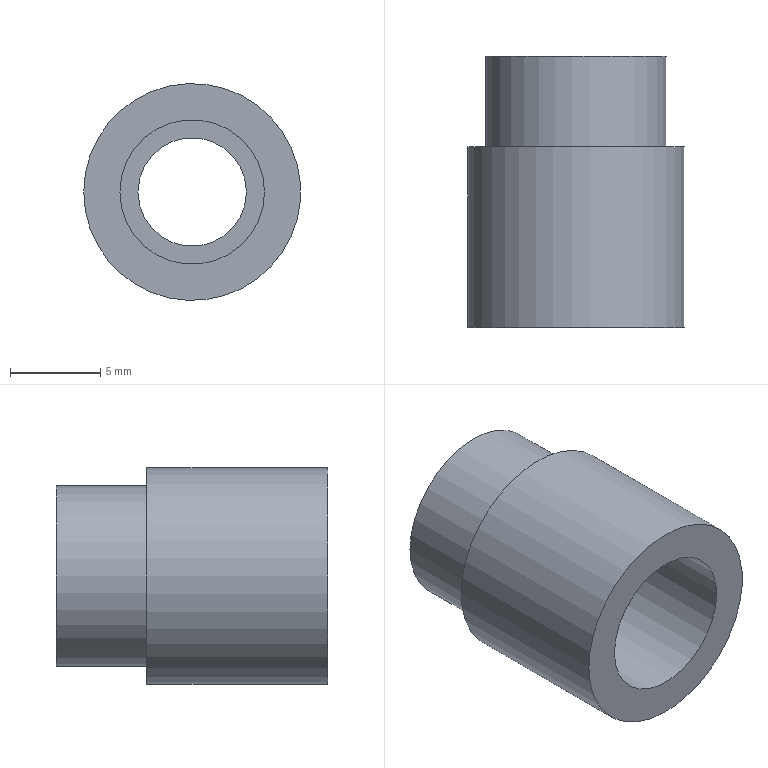Component | NX | 05D__27_2 | 1 solid | 8 faces | box 12 x 15 x 12 mm | volume 924 mm3 | cylinder 4 | plane 4 | commonest cylinder face diameters 6 x1 10 x1 12 x1 8 x1
STEP:
#1=CARTESIAN_POINT('',(0.,0.,0.));
#2=DIRECTION('',(0.,0.,1.));
#3=DIRECTION('',(1.,0.,0.));
#4=AXIS2_PLACEMENT_3D('',#1,#2,#3);
#5=CARTESIAN_POINT('',(63.522,90.09,209.432));
#6=VERTEX_POINT('',#5);
#7=CARTESIAN_POINT('',(66.522,90.09,209.432));
#8=DIRECTION('',(0.,1.,0.));
#9=DIRECTION('',(-1.,0.,0.));
#10=AXIS2_PLACEMENT_3D('',#7,#8,#9);
#11=CIRCLE('',#10,3.);
#12=CARTESIAN_POINT('',(66.522,90.09,209.432));
#13=DIRECTION('',(0.,1.,0.));
#14=DIRECTION('',(-1.,0.,0.));
#15=AXIS2_PLACEMENT_3D('',#12,#13,#14);
#16=CYLINDRICAL_SURFACE('',#15,3.);
#17=CARTESIAN_POINT('',(0.,0.));
#18=DIRECTION('',(1.,0.));
#19=VECTOR('',#18,1.);
#20=LINE('',#17,#19);
#21=(GEOMETRIC_REPRESENTATION_CONTEXT(2)PARAMETRIC_REPRESENTATION_CONTEXT()REPRESENTATION_CONTEXT('',''));
#22=DEFINITIONAL_REPRESENTATION('',(#20),#21);
#23=PCURVE('',#16,#22);
#24=CARTESIAN_POINT('',(66.522,90.09,212.432));
#25=DIRECTION('',(0.,1.,0.));
#26=DIRECTION('',(-1.,0.,0.));
#27=AXIS2_PLACEMENT_3D('',#24,#25,#26);
#28=PLANE('',#27);
#29=CARTESIAN_POINT('',(0.,-3.));
#30=DIRECTION('',(1.,0.));
#31=AXIS2_PLACEMENT_2D('',#29,#30);
#32=CIRCLE('',#31,3.);
#33=(GEOMETRIC_REPRESENTATION_CONTEXT(2)PARAMETRIC_REPRESENTATION_CONTEXT()REPRESENTATION_CONTEXT('',''));
#34=DEFINITIONAL_REPRESENTATION('',(#32),#33);
#35=PCURVE('',#28,#34);
#36=SURFACE_CURVE('',#11,(#23,#35),.PCURVE_S1.);
#37=EDGE_CURVE('',#6,#6,#36,.T.);
#38=ORIENTED_EDGE('',*,*,#37,.F.);
#39=CARTESIAN_POINT('',(63.522,83.09,209.432));
#40=VERTEX_POINT('',#39);
#41=CARTESIAN_POINT('',(63.522,83.09,209.432));
#42=CARTESIAN_POINT('',(63.522,90.09,209.432));
#43=B_SPLINE_CURVE_WITH_KNOTS('',1,(#41,#42),.UNSPECIFIED.,.F.,.F.,(2,2),(-7.,0.),.PIECEWISE_BEZIER_KNOTS.);
#44=CARTESIAN_POINT('',(0.,0.));
#45=DIRECTION('',(0.,1.));
#46=VECTOR('',#45,1.);
#47=LINE('',#44,#46);
#48=(GEOMETRIC_REPRESENTATION_CONTEXT(2)PARAMETRIC_REPRESENTATION_CONTEXT()REPRESENTATION_CONTEXT('',''));
#49=DEFINITIONAL_REPRESENTATION('',(#47),#48);
#50=PCURVE('',#16,#49);
#51=CARTESIAN_POINT('',(6.283,0.));
#52=DIRECTION('',(0.,1.));
#53=VECTOR('',#52,1.);
#54=LINE('',#51,#53);
#55=(GEOMETRIC_REPRESENTATION_CONTEXT(2)PARAMETRIC_REPRESENTATION_CONTEXT()REPRESENTATION_CONTEXT('',''));
#56=DEFINITIONAL_REPRESENTATION('',(#54),#55);
#57=PCURVE('',#16,#56);
#58=SEAM_CURVE('',#43,(#50,#57),.PCURVE_S1.);
#59=EDGE_CURVE('',#40,#6,#58,.T.);
#60=ORIENTED_EDGE('',*,*,#59,.F.);
#61=CARTESIAN_POINT('',(66.522,83.09,209.432));
#62=DIRECTION('',(0.,1.,0.));
#63=DIRECTION('',(-1.,0.,0.));
#64=AXIS2_PLACEMENT_3D('',#61,#62,#63);
#65=CIRCLE('',#64,3.);
#66=CARTESIAN_POINT('',(0.,-7.));
#67=DIRECTION('',(1.,0.));
#68=VECTOR('',#67,1.);
#69=LINE('',#66,#68);
#70=(GEOMETRIC_REPRESENTATION_CONTEXT(2)PARAMETRIC_REPRESENTATION_CONTEXT()REPRESENTATION_CONTEXT('',''));
#71=DEFINITIONAL_REPRESENTATION('',(#69),#70);
#72=PCURVE('',#16,#71);
#73=CARTESIAN_POINT('',(66.522,83.09,213.432));
#74=DIRECTION('',(0.,-1.,-0.));
#75=DIRECTION('',(1.,0.,0.));
#76=AXIS2_PLACEMENT_3D('',#73,#74,#75);
#77=PLANE('',#76);
#78=CARTESIAN_POINT('',(-3.,-4.));
#79=CARTESIAN_POINT('',(-3.,1.196));
#80=CARTESIAN_POINT('',(1.5,-1.402));
#81=CARTESIAN_POINT('',(6.,-4.));
#82=CARTESIAN_POINT('',(1.5,-6.598));
#83=CARTESIAN_POINT('',(-3.,-9.196));
#84=CARTESIAN_POINT('',(-3.,-4.));
#85=(BOUNDED_CURVE()B_SPLINE_CURVE(2,(#78,#79,#80,#81,#82,#83,#84),.UNSPECIFIED.,.T.,.F.)B_SPLINE_CURVE_WITH_KNOTS((1,2,2,2,2,1),(-2.094,0.,2.094,4.189,6.283,8.378),.UNSPECIFIED.)CURVE()GEOMETRIC_REPRESENTATION_ITEM()RATIONAL_B_SPLINE_CURVE((1.,0.5,1.,0.5,1.,0.5,1.))REPRESENTATION_ITEM(''));
#86=(GEOMETRIC_REPRESENTATION_CONTEXT(2)PARAMETRIC_REPRESENTATION_CONTEXT()REPRESENTATION_CONTEXT('',''));
#87=DEFINITIONAL_REPRESENTATION('',(#85),#86);
#88=PCURVE('',#77,#87);
#89=SURFACE_CURVE('',#65,(#72,#88),.PCURVE_S1.);
#90=EDGE_CURVE('',#40,#40,#89,.T.);
#91=ORIENTED_EDGE('',*,*,#90,.T.);
#92=ORIENTED_EDGE('',*,*,#59,.T.);
#93=EDGE_LOOP('',(#38,#60,#91,#92));
#94=FACE_BOUND('',#93,.F.);
#95=ADVANCED_FACE('',(#94),#16,.F.);
#96=CARTESIAN_POINT('',(61.522,90.09,209.432));
#97=VERTEX_POINT('',#96);
#98=CARTESIAN_POINT('',(66.522,90.09,209.432));
#99=DIRECTION('',(0.,1.,0.));
#100=DIRECTION('',(-1.,0.,0.));
#101=AXIS2_PLACEMENT_3D('',#98,#99,#100);
#102=CIRCLE('',#101,5.);
#103=CARTESIAN_POINT('',(0.,-3.));
#104=DIRECTION('',(1.,0.));
#105=AXIS2_PLACEMENT_2D('',#103,#104);
#106=CIRCLE('',#105,5.);
#107=(GEOMETRIC_REPRESENTATION_CONTEXT(2)PARAMETRIC_REPRESENTATION_CONTEXT()REPRESENTATION_CONTEXT('',''));
#108=DEFINITIONAL_REPRESENTATION('',(#106),#107);
#109=PCURVE('',#28,#108);
#110=CARTESIAN_POINT('',(66.522,90.09,209.432));
#111=DIRECTION('',(0.,1.,0.));
#112=DIRECTION('',(-1.,0.,0.));
#113=AXIS2_PLACEMENT_3D('',#110,#111,#112);
#114=CYLINDRICAL_SURFACE('',#113,5.);
#115=CARTESIAN_POINT('',(0.,0.));
#116=DIRECTION('',(1.,0.));
#117=VECTOR('',#116,1.);
#118=LINE('',#115,#117);
#119=(GEOMETRIC_REPRESENTATION_CONTEXT(2)PARAMETRIC_REPRESENTATION_CONTEXT()REPRESENTATION_CONTEXT('',''));
#120=DEFINITIONAL_REPRESENTATION('',(#118),#119);
#121=PCURVE('',#114,#120);
#122=SURFACE_CURVE('',#102,(#109,#121),.PCURVE_S1.);
#123=EDGE_CURVE('',#97,#97,#122,.T.);
#124=ORIENTED_EDGE('',*,*,#123,.T.);
#125=EDGE_LOOP('',(#124));
#126=FACE_BOUND('',#125,.T.);
#127=ORIENTED_EDGE('',*,*,#37,.F.);
#128=EDGE_LOOP('',(#127));
#129=FACE_BOUND('',#128,.T.);
#130=ADVANCED_FACE('',(#126,#129),#28,.T.);
#131=CARTESIAN_POINT('',(61.522,85.09,209.432));
#132=VERTEX_POINT('',#131);
#133=CARTESIAN_POINT('',(66.522,85.09,209.432));
#134=DIRECTION('',(0.,1.,0.));
#135=DIRECTION('',(-1.,0.,0.));
#136=AXIS2_PLACEMENT_3D('',#133,#134,#135);
#137=CIRCLE('',#136,5.);
#138=CARTESIAN_POINT('',(0.,-5.));
#139=DIRECTION('',(1.,0.));
#140=VECTOR('',#139,1.);
#141=LINE('',#138,#140);
#142=(GEOMETRIC_REPRESENTATION_CONTEXT(2)PARAMETRIC_REPRESENTATION_CONTEXT()REPRESENTATION_CONTEXT('',''));
#143=DEFINITIONAL_REPRESENTATION('',(#141),#142);
#144=PCURVE('',#114,#143);
#145=CARTESIAN_POINT('',(66.522,85.09,214.432));
#146=DIRECTION('',(0.,1.,0.));
#147=DIRECTION('',(-1.,0.,0.));
#148=AXIS2_PLACEMENT_3D('',#145,#146,#147);
#149=PLANE('',#148);
#150=CARTESIAN_POINT('',(0.,-5.));
#151=DIRECTION('',(1.,0.));
#152=AXIS2_PLACEMENT_2D('',#150,#151);
#153=CIRCLE('',#152,5.);
#154=(GEOMETRIC_REPRESENTATION_CONTEXT(2)PARAMETRIC_REPRESENTATION_CONTEXT()REPRESENTATION_CONTEXT('',''));
#155=DEFINITIONAL_REPRESENTATION('',(#153),#154);
#156=PCURVE('',#149,#155);
#157=SURFACE_CURVE('',#137,(#144,#156),.PCURVE_S1.);
#158=EDGE_CURVE('',#132,#132,#157,.T.);
#159=ORIENTED_EDGE('',*,*,#158,.T.);
#160=CARTESIAN_POINT('',(61.522,85.09,209.432));
#161=CARTESIAN_POINT('',(61.522,90.09,209.432));
#162=B_SPLINE_CURVE_WITH_KNOTS('',1,(#160,#161),.UNSPECIFIED.,.F.,.F.,(2,2),(-5.,0.),.PIECEWISE_BEZIER_KNOTS.);
#163=CARTESIAN_POINT('',(6.283,0.));
#164=DIRECTION('',(0.,1.));
#165=VECTOR('',#164,1.);
#166=LINE('',#163,#165);
#167=(GEOMETRIC_REPRESENTATION_CONTEXT(2)PARAMETRIC_REPRESENTATION_CONTEXT()REPRESENTATION_CONTEXT('',''));
#168=DEFINITIONAL_REPRESENTATION('',(#166),#167);
#169=PCURVE('',#114,#168);
#170=CARTESIAN_POINT('',(0.,0.));
#171=DIRECTION('',(0.,1.));
#172=VECTOR('',#171,1.);
#173=LINE('',#170,#172);
#174=(GEOMETRIC_REPRESENTATION_CONTEXT(2)PARAMETRIC_REPRESENTATION_CONTEXT()REPRESENTATION_CONTEXT('',''));
#175=DEFINITIONAL_REPRESENTATION('',(#173),#174);
#176=PCURVE('',#114,#175);
#177=SEAM_CURVE('',#162,(#169,#176),.PCURVE_S1.);
#178=EDGE_CURVE('',#132,#97,#177,.T.);
#179=ORIENTED_EDGE('',*,*,#178,.T.);
#180=ORIENTED_EDGE('',*,*,#123,.F.);
#181=ORIENTED_EDGE('',*,*,#178,.F.);
#182=EDGE_LOOP('',(#159,#179,#180,#181));
#183=FACE_BOUND('',#182,.T.);
#184=ADVANCED_FACE('',(#183),#114,.T.);
#185=CARTESIAN_POINT('',(60.522,85.09,209.432));
#186=VERTEX_POINT('',#185);
#187=CARTESIAN_POINT('',(66.522,85.09,209.432));
#188=DIRECTION('',(0.,1.,0.));
#189=DIRECTION('',(-1.,0.,0.));
#190=AXIS2_PLACEMENT_3D('',#187,#188,#189);
#191=CIRCLE('',#190,6.);
#192=CARTESIAN_POINT('',(0.,-5.));
#193=DIRECTION('',(1.,0.));
#194=AXIS2_PLACEMENT_2D('',#192,#193);
#195=CIRCLE('',#194,6.);
#196=(GEOMETRIC_REPRESENTATION_CONTEXT(2)PARAMETRIC_REPRESENTATION_CONTEXT()REPRESENTATION_CONTEXT('',''));
#197=DEFINITIONAL_REPRESENTATION('',(#195),#196);
#198=PCURVE('',#149,#197);
#199=CARTESIAN_POINT('',(66.522,90.09,209.432));
#200=DIRECTION('',(0.,1.,0.));
#201=DIRECTION('',(-1.,0.,0.));
#202=AXIS2_PLACEMENT_3D('',#199,#200,#201);
#203=CYLINDRICAL_SURFACE('',#202,6.);
#204=CARTESIAN_POINT('',(0.,-5.));
#205=DIRECTION('',(1.,0.));
#206=VECTOR('',#205,1.);
#207=LINE('',#204,#206);
#208=(GEOMETRIC_REPRESENTATION_CONTEXT(2)PARAMETRIC_REPRESENTATION_CONTEXT()REPRESENTATION_CONTEXT('',''));
#209=DEFINITIONAL_REPRESENTATION('',(#207),#208);
#210=PCURVE('',#203,#209);
#211=SURFACE_CURVE('',#191,(#198,#210),.PCURVE_S1.);
#212=EDGE_CURVE('',#186,#186,#211,.T.);
#213=ORIENTED_EDGE('',*,*,#212,.T.);
#214=EDGE_LOOP('',(#213));
#215=FACE_BOUND('',#214,.T.);
#216=ORIENTED_EDGE('',*,*,#158,.F.);
#217=EDGE_LOOP('',(#216));
#218=FACE_BOUND('',#217,.T.);
#219=ADVANCED_FACE('',(#215,#218),#149,.T.);
#220=CARTESIAN_POINT('',(60.522,75.09,209.432));
#221=VERTEX_POINT('',#220);
#222=CARTESIAN_POINT('',(66.522,75.09,209.432));
#223=DIRECTION('',(0.,1.,0.));
#224=DIRECTION('',(-1.,0.,0.));
#225=AXIS2_PLACEMENT_3D('',#222,#223,#224);
#226=CIRCLE('',#225,6.);
#227=CARTESIAN_POINT('',(0.,-15.));
#228=DIRECTION('',(1.,0.));
#229=VECTOR('',#228,1.);
#230=LINE('',#227,#229);
#231=(GEOMETRIC_REPRESENTATION_CONTEXT(2)PARAMETRIC_REPRESENTATION_CONTEXT()REPRESENTATION_CONTEXT('',''));
#232=DEFINITIONAL_REPRESENTATION('',(#230),#231);
#233=PCURVE('',#203,#232);
#234=CARTESIAN_POINT('',(66.522,75.09,215.432));
#235=DIRECTION('',(0.,-1.,-0.));
#236=DIRECTION('',(1.,0.,0.));
#237=AXIS2_PLACEMENT_3D('',#234,#235,#236);
#238=PLANE('',#237);
#239=CARTESIAN_POINT('',(-6.,-6.));
#240=CARTESIAN_POINT('',(-6.,4.392));
#241=CARTESIAN_POINT('',(3.,-0.8038));
#242=CARTESIAN_POINT('',(12.,-6.));
#243=CARTESIAN_POINT('',(3.,-11.196));
#244=CARTESIAN_POINT('',(-6.,-16.392));
#245=CARTESIAN_POINT('',(-6.,-6.));
#246=(BOUNDED_CURVE()B_SPLINE_CURVE(2,(#239,#240,#241,#242,#243,#244,#245),.UNSPECIFIED.,.T.,.F.)B_SPLINE_CURVE_WITH_KNOTS((1,2,2,2,2,1),(-2.094,0.,2.094,4.189,6.283,8.378),.UNSPECIFIED.)CURVE()GEOMETRIC_REPRESENTATION_ITEM()RATIONAL_B_SPLINE_CURVE((1.,0.5,1.,0.5,1.,0.5,1.))REPRESENTATION_ITEM(''));
#247=(GEOMETRIC_REPRESENTATION_CONTEXT(2)PARAMETRIC_REPRESENTATION_CONTEXT()REPRESENTATION_CONTEXT('',''));
#248=DEFINITIONAL_REPRESENTATION('',(#246),#247);
#249=PCURVE('',#238,#248);
#250=SURFACE_CURVE('',#226,(#233,#249),.PCURVE_S1.);
#251=EDGE_CURVE('',#221,#221,#250,.T.);
#252=ORIENTED_EDGE('',*,*,#251,.T.);
#253=CARTESIAN_POINT('',(60.522,75.09,209.432));
#254=CARTESIAN_POINT('',(60.522,85.09,209.432));
#255=B_SPLINE_CURVE_WITH_KNOTS('',1,(#253,#254),.UNSPECIFIED.,.F.,.F.,(2,2),(-15.,-5.),.PIECEWISE_BEZIER_KNOTS.);
#256=CARTESIAN_POINT('',(6.283,0.));
#257=DIRECTION('',(0.,1.));
#258=VECTOR('',#257,1.);
#259=LINE('',#256,#258);
#260=(GEOMETRIC_REPRESENTATION_CONTEXT(2)PARAMETRIC_REPRESENTATION_CONTEXT()REPRESENTATION_CONTEXT('',''));
#261=DEFINITIONAL_REPRESENTATION('',(#259),#260);
#262=PCURVE('',#203,#261);
#263=CARTESIAN_POINT('',(0.,0.));
#264=DIRECTION('',(0.,1.));
#265=VECTOR('',#264,1.);
#266=LINE('',#263,#265);
#267=(GEOMETRIC_REPRESENTATION_CONTEXT(2)PARAMETRIC_REPRESENTATION_CONTEXT()REPRESENTATION_CONTEXT('',''));
#268=DEFINITIONAL_REPRESENTATION('',(#266),#267);
#269=PCURVE('',#203,#268);
#270=SEAM_CURVE('',#255,(#262,#269),.PCURVE_S1.);
#271=EDGE_CURVE('',#221,#186,#270,.T.);
#272=ORIENTED_EDGE('',*,*,#271,.T.);
#273=ORIENTED_EDGE('',*,*,#212,.F.);
#274=ORIENTED_EDGE('',*,*,#271,.F.);
#275=EDGE_LOOP('',(#252,#272,#273,#274));
#276=FACE_BOUND('',#275,.T.);
#277=ADVANCED_FACE('',(#276),#203,.T.);
#278=CARTESIAN_POINT('',(62.522,75.09,209.432));
#279=VERTEX_POINT('',#278);
#280=CARTESIAN_POINT('',(66.522,75.09,209.432));
#281=DIRECTION('',(0.,1.,0.));
#282=DIRECTION('',(-1.,0.,0.));
#283=AXIS2_PLACEMENT_3D('',#280,#281,#282);
#284=CIRCLE('',#283,4.);
#285=CARTESIAN_POINT('',(-4.,-6.));
#286=CARTESIAN_POINT('',(-4.,0.9282));
#287=CARTESIAN_POINT('',(2.,-2.536));
#288=CARTESIAN_POINT('',(8.,-6.));
#289=CARTESIAN_POINT('',(2.,-9.464));
#290=CARTESIAN_POINT('',(-4.,-12.928));
#291=CARTESIAN_POINT('',(-4.,-6.));
#292=(BOUNDED_CURVE()B_SPLINE_CURVE(2,(#285,#286,#287,#288,#289,#290,#291),.UNSPECIFIED.,.T.,.F.)B_SPLINE_CURVE_WITH_KNOTS((1,2,2,2,2,1),(-2.094,0.,2.094,4.189,6.283,8.378),.UNSPECIFIED.)CURVE()GEOMETRIC_REPRESENTATION_ITEM()RATIONAL_B_SPLINE_CURVE((1.,0.5,1.,0.5,1.,0.5,1.))REPRESENTATION_ITEM(''));
#293=(GEOMETRIC_REPRESENTATION_CONTEXT(2)PARAMETRIC_REPRESENTATION_CONTEXT()REPRESENTATION_CONTEXT('',''));
#294=DEFINITIONAL_REPRESENTATION('',(#292),#293);
#295=PCURVE('',#238,#294);
#296=CARTESIAN_POINT('',(66.522,90.09,209.432));
#297=DIRECTION('',(0.,1.,0.));
#298=DIRECTION('',(-1.,0.,0.));
#299=AXIS2_PLACEMENT_3D('',#296,#297,#298);
#300=CYLINDRICAL_SURFACE('',#299,4.);
#301=CARTESIAN_POINT('',(0.,-15.));
#302=DIRECTION('',(1.,0.));
#303=VECTOR('',#302,1.);
#304=LINE('',#301,#303);
#305=(GEOMETRIC_REPRESENTATION_CONTEXT(2)PARAMETRIC_REPRESENTATION_CONTEXT()REPRESENTATION_CONTEXT('',''));
#306=DEFINITIONAL_REPRESENTATION('',(#304),#305);
#307=PCURVE('',#300,#306);
#308=SURFACE_CURVE('',#284,(#295,#307),.PCURVE_S1.);
#309=EDGE_CURVE('',#279,#279,#308,.T.);
#310=ORIENTED_EDGE('',*,*,#309,.T.);
#311=EDGE_LOOP('',(#310));
#312=FACE_BOUND('',#311,.T.);
#313=ORIENTED_EDGE('',*,*,#251,.F.);
#314=EDGE_LOOP('',(#313));
#315=FACE_BOUND('',#314,.T.);
#316=ADVANCED_FACE('',(#312,#315),#238,.T.);
#317=CARTESIAN_POINT('',(62.522,83.09,209.432));
#318=VERTEX_POINT('',#317);
#319=CARTESIAN_POINT('',(66.522,83.09,209.432));
#320=DIRECTION('',(0.,1.,0.));
#321=DIRECTION('',(-1.,0.,0.));
#322=AXIS2_PLACEMENT_3D('',#319,#320,#321);
#323=CIRCLE('',#322,4.);
#324=CARTESIAN_POINT('',(0.,-7.));
#325=DIRECTION('',(1.,0.));
#326=VECTOR('',#325,1.);
#327=LINE('',#324,#326);
#328=(GEOMETRIC_REPRESENTATION_CONTEXT(2)PARAMETRIC_REPRESENTATION_CONTEXT()REPRESENTATION_CONTEXT('',''));
#329=DEFINITIONAL_REPRESENTATION('',(#327),#328);
#330=PCURVE('',#300,#329);
#331=CARTESIAN_POINT('',(-4.,-4.));
#332=CARTESIAN_POINT('',(-4.,2.928));
#333=CARTESIAN_POINT('',(2.,-0.5359));
#334=CARTESIAN_POINT('',(8.,-4.));
#335=CARTESIAN_POINT('',(2.,-7.464));
#336=CARTESIAN_POINT('',(-4.,-10.928));
#337=CARTESIAN_POINT('',(-4.,-4.));
#338=(BOUNDED_CURVE()B_SPLINE_CURVE(2,(#331,#332,#333,#334,#335,#336,#337),.UNSPECIFIED.,.T.,.F.)B_SPLINE_CURVE_WITH_KNOTS((1,2,2,2,2,1),(-2.094,0.,2.094,4.189,6.283,8.378),.UNSPECIFIED.)CURVE()GEOMETRIC_REPRESENTATION_ITEM()RATIONAL_B_SPLINE_CURVE((1.,0.5,1.,0.5,1.,0.5,1.))REPRESENTATION_ITEM(''));
#339=(GEOMETRIC_REPRESENTATION_CONTEXT(2)PARAMETRIC_REPRESENTATION_CONTEXT()REPRESENTATION_CONTEXT('',''));
#340=DEFINITIONAL_REPRESENTATION('',(#338),#339);
#341=PCURVE('',#77,#340);
#342=SURFACE_CURVE('',#323,(#330,#341),.PCURVE_S1.);
#343=EDGE_CURVE('',#318,#318,#342,.T.);
#344=ORIENTED_EDGE('',*,*,#343,.F.);
#345=CARTESIAN_POINT('',(62.522,75.09,209.432));
#346=CARTESIAN_POINT('',(62.522,83.09,209.432));
#347=B_SPLINE_CURVE_WITH_KNOTS('',1,(#345,#346),.UNSPECIFIED.,.F.,.F.,(2,2),(-15.,-7.),.PIECEWISE_BEZIER_KNOTS.);
#348=CARTESIAN_POINT('',(0.,0.));
#349=DIRECTION('',(0.,1.));
#350=VECTOR('',#349,1.);
#351=LINE('',#348,#350);
#352=(GEOMETRIC_REPRESENTATION_CONTEXT(2)PARAMETRIC_REPRESENTATION_CONTEXT()REPRESENTATION_CONTEXT('',''));
#353=DEFINITIONAL_REPRESENTATION('',(#351),#352);
#354=PCURVE('',#300,#353);
#355=CARTESIAN_POINT('',(6.283,0.));
#356=DIRECTION('',(0.,1.));
#357=VECTOR('',#356,1.);
#358=LINE('',#355,#357);
#359=(GEOMETRIC_REPRESENTATION_CONTEXT(2)PARAMETRIC_REPRESENTATION_CONTEXT()REPRESENTATION_CONTEXT('',''));
#360=DEFINITIONAL_REPRESENTATION('',(#358),#359);
#361=PCURVE('',#300,#360);
#362=SEAM_CURVE('',#347,(#354,#361),.PCURVE_S1.);
#363=EDGE_CURVE('',#279,#318,#362,.T.);
#364=ORIENTED_EDGE('',*,*,#363,.F.);
#365=ORIENTED_EDGE('',*,*,#309,.T.);
#366=ORIENTED_EDGE('',*,*,#363,.T.);
#367=EDGE_LOOP('',(#344,#364,#365,#366));
#368=FACE_BOUND('',#367,.F.);
#369=ADVANCED_FACE('',(#368),#300,.F.);
#370=ORIENTED_EDGE('',*,*,#90,.T.);
#371=EDGE_LOOP('',(#370));
#372=FACE_BOUND('',#371,.T.);
#373=ORIENTED_EDGE('',*,*,#343,.F.);
#374=EDGE_LOOP('',(#373));
#375=FACE_BOUND('',#374,.T.);
#376=ADVANCED_FACE('',(#372,#375),#77,.T.);
#377=CLOSED_SHELL('',(#95,#130,#184,#219,#277,#316,#369,#376));
#378=MANIFOLD_SOLID_BREP('',#377);
#379=(LENGTH_UNIT()NAMED_UNIT(*)SI_UNIT(.MILLI.,.METRE.));
#380=UNCERTAINTY_MEASURE_WITH_UNIT(LENGTH_MEASURE(0.00001),#379,'','');
#381=(NAMED_UNIT(*)PLANE_ANGLE_UNIT()SI_UNIT($,.RADIAN.));
#382=(NAMED_UNIT(*)SI_UNIT($,.STERADIAN.)SOLID_ANGLE_UNIT());
#383=(GEOMETRIC_REPRESENTATION_CONTEXT(3)GLOBAL_UNCERTAINTY_ASSIGNED_CONTEXT((#380))GLOBAL_UNIT_ASSIGNED_CONTEXT((#379,#381,#382))REPRESENTATION_CONTEXT('',''));
#384=ADVANCED_BREP_SHAPE_REPRESENTATION('',(#4,#378),#383);